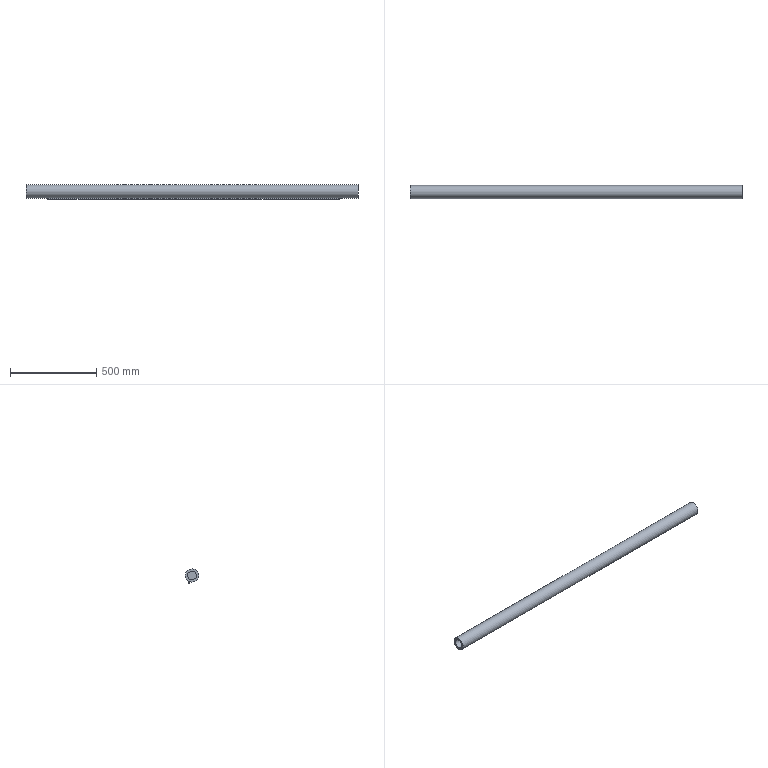Component | NX | CYL_BODY_2 | 2 solids | 12 faces | volume 4939040 mm3 | plane 5 | spline 5 | cylinder 2 | commonest cylinder face diameters 76.2 x1 51 x1